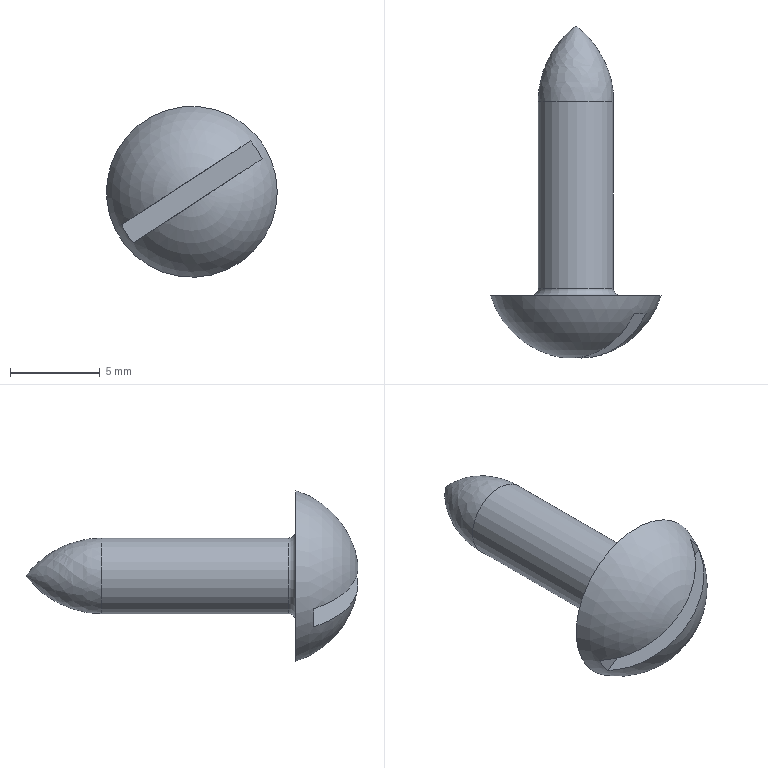Component | NX | 7_HALF_ROUND_SCREW_M5X15 | 1 solid | 8 faces | box 9.5 x 18.46 x 9.5 mm | volume 312 mm3 | plane 4 | sphere 1 | cylinder 1 | spline 1 | torus 1 | commonest cylinder face diameters 4.2 x1
STEP:
#1=CARTESIAN_POINT('',(0.,0.,0.));
#2=DIRECTION('',(0.,0.,1.));
#3=DIRECTION('',(1.,0.,0.));
#4=AXIS2_PLACEMENT_3D('',#1,#2,#3);
#5=CARTESIAN_POINT('',(-55.107,-157.206,-235.621));
#6=VERTEX_POINT('',#5);
#7=CARTESIAN_POINT('',(-55.507,-157.206,-235.093));
#8=VERTEX_POINT('',#7);
#9=CARTESIAN_POINT('',(-59.084,-157.206,-238.219));
#10=DIRECTION('',(0.,-1.,0.));
#11=DIRECTION('',(0.8372,0.,0.5469));
#12=AXIS2_PLACEMENT_3D('',#9,#10,#11);
#13=CIRCLE('',#12,4.75);
#14=CARTESIAN_POINT('',(-59.084,-155.733,-238.219));
#15=DIRECTION('',(0.,-1.,0.));
#16=DIRECTION('',(-0.5469,0.,0.8372));
#17=AXIS2_PLACEMENT_3D('',#14,#15,#16);
#18=SPHERICAL_SURFACE('',#17,4.973);
#19=CARTESIAN_POINT('',(10.996,0.3007));
#20=CARTESIAN_POINT('',(11.091,0.3007));
#21=CARTESIAN_POINT('',(11.281,0.3007));
#22=CARTESIAN_POINT('',(11.567,0.3007));
#23=CARTESIAN_POINT('',(11.852,0.3007));
#24=CARTESIAN_POINT('',(12.138,0.3007));
#25=CARTESIAN_POINT('',(12.424,0.3007));
#26=CARTESIAN_POINT('',(12.709,0.3007));
#27=CARTESIAN_POINT('',(12.995,0.3007));
#28=CARTESIAN_POINT('',(13.28,0.3007));
#29=CARTESIAN_POINT('',(13.566,0.3007));
#30=CARTESIAN_POINT('',(13.852,0.3007));
#31=CARTESIAN_POINT('',(14.137,0.3007));
#32=CARTESIAN_POINT('',(14.423,0.3007));
#33=CARTESIAN_POINT('',(14.708,0.3007));
#34=CARTESIAN_POINT('',(14.994,0.3007));
#35=CARTESIAN_POINT('',(15.28,0.3007));
#36=CARTESIAN_POINT('',(15.565,0.3007));
#37=CARTESIAN_POINT('',(15.851,0.3007));
#38=CARTESIAN_POINT('',(16.136,0.3007));
#39=CARTESIAN_POINT('',(16.422,0.3007));
#40=CARTESIAN_POINT('',(16.708,0.3007));
#41=CARTESIAN_POINT('',(16.993,0.3007));
#42=CARTESIAN_POINT('',(17.184,0.3007));
#43=CARTESIAN_POINT('',(17.279,0.3007));
#44=B_SPLINE_CURVE_WITH_KNOTS('',3,(#19,#20,#21,#22,#23,#24,#25,#26,#27,#28,#29,#30,#31,#32,#33,#34,#35,#36,#37,#38,#39,#40,#41,#42,#43),.UNSPECIFIED.,.F.,.F.,(4,1,1,1,1,1,1,1,1,1,1,1,1,1,1,1,1,1,1,1,1,1,4),(0.,0.2856,0.5712,0.8568,1.142,1.428,1.714,1.999,2.285,2.57,2.856,3.142,3.427,3.713,3.998,4.284,4.57,4.855,5.141,5.426,5.712,5.998,6.283),.QUASI_UNIFORM_KNOTS.);
#45=(GEOMETRIC_REPRESENTATION_CONTEXT(2)PARAMETRIC_REPRESENTATION_CONTEXT()REPRESENTATION_CONTEXT('',''));
#46=DEFINITIONAL_REPRESENTATION('',(#44),#45);
#47=PCURVE('',#18,#46);
#48=CARTESIAN_POINT('',(-60.232,-157.206,-236.461));
#49=DIRECTION('',(0.,-1.,0.));
#50=DIRECTION('',(0.8372,0.,0.5469));
#51=AXIS2_PLACEMENT_3D('',#48,#49,#50);
#52=PLANE('',#51);
#53=CARTESIAN_POINT('',(-0.,-2.1));
#54=DIRECTION('',(1.,-0.));
#55=AXIS2_PLACEMENT_2D('',#53,#54);
#56=CIRCLE('',#55,4.75);
#57=(GEOMETRIC_REPRESENTATION_CONTEXT(2)PARAMETRIC_REPRESENTATION_CONTEXT()REPRESENTATION_CONTEXT('',''));
#58=DEFINITIONAL_REPRESENTATION('',(#56),#57);
#59=PCURVE('',#52,#58);
#60=SURFACE_CURVE('',#13,(#47,#59),.PCURVE_S1.);
#61=EDGE_CURVE('',#6,#8,#60,.T.);
#62=ORIENTED_EDGE('',*,*,#61,.T.);
#63=CARTESIAN_POINT('',(-55.835,-158.206,-235.38));
#64=VERTEX_POINT('',#63);
#65=CARTESIAN_POINT('',(-55.507,-157.206,-235.093));
#66=CARTESIAN_POINT('',(-55.568,-157.467,-235.147));
#67=CARTESIAN_POINT('',(-55.643,-157.722,-235.212));
#68=CARTESIAN_POINT('',(-55.733,-157.969,-235.29));
#69=CARTESIAN_POINT('',(-55.835,-158.206,-235.38));
#70=B_SPLINE_CURVE_WITH_KNOTS('',4,(#65,#66,#67,#68,#69),.UNSPECIFIED.,.F.,.F.,(5,5),(0.3007,0.5205),.PIECEWISE_BEZIER_KNOTS.);
#71=CARTESIAN_POINT('',(11.135,0.));
#72=DIRECTION('',(0.,1.));
#73=VECTOR('',#72,1.);
#74=LINE('',#71,#73);
#75=(GEOMETRIC_REPRESENTATION_CONTEXT(2)PARAMETRIC_REPRESENTATION_CONTEXT()REPRESENTATION_CONTEXT('',''));
#76=DEFINITIONAL_REPRESENTATION('',(#74),#75);
#77=PCURVE('',#18,#76);
#78=CARTESIAN_POINT('',(4.852,0.));
#79=DIRECTION('',(0.,1.));
#80=VECTOR('',#79,1.);
#81=LINE('',#78,#80);
#82=(GEOMETRIC_REPRESENTATION_CONTEXT(2)PARAMETRIC_REPRESENTATION_CONTEXT()REPRESENTATION_CONTEXT('',''));
#83=DEFINITIONAL_REPRESENTATION('',(#81),#82);
#84=PCURVE('',#18,#83);
#85=SEAM_CURVE('',#70,(#77,#84),.PCURVE_S1.);
#86=EDGE_CURVE('',#8,#64,#85,.T.);
#87=ORIENTED_EDGE('',*,*,#86,.T.);
#88=CARTESIAN_POINT('',(-55.179,-158.206,-236.384));
#89=VERTEX_POINT('',#88);
#90=CARTESIAN_POINT('',(-59.084,-158.206,-238.219));
#91=DIRECTION('',(0.,-1.,0.));
#92=DIRECTION('',(0.8372,0.,0.5469));
#93=AXIS2_PLACEMENT_3D('',#90,#91,#92);
#94=CIRCLE('',#93,4.315);
#95=CARTESIAN_POINT('',(4.712,0.5205));
#96=DIRECTION('',(1.,0.));
#97=VECTOR('',#96,1.);
#98=LINE('',#95,#97);
#99=(GEOMETRIC_REPRESENTATION_CONTEXT(2)PARAMETRIC_REPRESENTATION_CONTEXT()REPRESENTATION_CONTEXT('',''));
#100=DEFINITIONAL_REPRESENTATION('',(#98),#99);
#101=PCURVE('',#18,#100);
#102=CARTESIAN_POINT('',(-51.131,-158.206,-233.023));
#103=DIRECTION('',(0.,-1.,0.));
#104=DIRECTION('',(0.8372,0.,0.5469));
#105=AXIS2_PLACEMENT_3D('',#102,#103,#104);
#106=PLANE('',#105);
#107=CARTESIAN_POINT('',(-9.5,-0.));
#108=DIRECTION('',(1.,-0.));
#109=AXIS2_PLACEMENT_2D('',#107,#108);
#110=CIRCLE('',#109,4.315);
#111=(GEOMETRIC_REPRESENTATION_CONTEXT(2)PARAMETRIC_REPRESENTATION_CONTEXT()REPRESENTATION_CONTEXT('',''));
#112=DEFINITIONAL_REPRESENTATION('',(#110),#111);
#113=PCURVE('',#106,#112);
#114=SURFACE_CURVE('',#94,(#101,#113),.PCURVE_S1.);
#115=EDGE_CURVE('',#89,#64,#114,.T.);
#116=ORIENTED_EDGE('',*,*,#115,.F.);
#117=CARTESIAN_POINT('',(-62.333,-158.206,-241.058));
#118=VERTEX_POINT('',#117);
#119=CARTESIAN_POINT('',(-58.756,-155.733,-238.721));
#120=DIRECTION('',(-0.5469,0.,0.8372));
#121=DIRECTION('',(-0.,-1.,0.));
#122=AXIS2_PLACEMENT_3D('',#119,#120,#121);
#123=CIRCLE('',#122,4.937);
#124=CARTESIAN_POINT('',(7.993,0.5205));
#125=CARTESIAN_POINT('',(7.996,0.5519));
#126=CARTESIAN_POINT('',(8.002,0.6146));
#127=CARTESIAN_POINT('',(8.013,0.7086));
#128=CARTESIAN_POINT('',(8.028,0.8024));
#129=CARTESIAN_POINT('',(8.047,0.8959));
#130=CARTESIAN_POINT('',(8.074,0.989));
#131=CARTESIAN_POINT('',(8.111,1.081));
#132=CARTESIAN_POINT('',(8.165,1.173));
#133=CARTESIAN_POINT('',(8.25,1.262));
#134=CARTESIAN_POINT('',(8.404,1.347));
#135=CARTESIAN_POINT('',(8.685,1.423));
#136=CARTESIAN_POINT('',(9.425,1.463));
#137=CARTESIAN_POINT('',(10.164,1.423));
#138=CARTESIAN_POINT('',(10.445,1.347));
#139=CARTESIAN_POINT('',(10.6,1.262));
#140=CARTESIAN_POINT('',(10.684,1.173));
#141=CARTESIAN_POINT('',(10.739,1.081));
#142=CARTESIAN_POINT('',(10.776,0.989));
#143=CARTESIAN_POINT('',(10.802,0.8959));
#144=CARTESIAN_POINT('',(10.822,0.8024));
#145=CARTESIAN_POINT('',(10.837,0.7086));
#146=CARTESIAN_POINT('',(10.848,0.6146));
#147=CARTESIAN_POINT('',(10.854,0.5519));
#148=CARTESIAN_POINT('',(10.856,0.5205));
#149=B_SPLINE_CURVE_WITH_KNOTS('',3,(#124,#125,#126,#127,#128,#129,#130,#131,#132,#133,#134,#135,#136,#137,#138,#139,#140,#141,#142,#143,#144,#145,#146,#147,#148),.UNSPECIFIED.,.F.,.F.,(4,1,1,1,1,1,1,1,1,1,1,1,1,1,1,1,1,1,1,1,1,1,4),(5.237,5.332,5.427,5.522,5.617,5.713,5.808,5.903,5.998,6.093,6.188,6.283,6.378,6.473,6.568,6.664,6.759,6.854,6.949,7.044,7.139,7.234,7.329),.QUASI_UNIFORM_KNOTS.);
#150=(GEOMETRIC_REPRESENTATION_CONTEXT(2)PARAMETRIC_REPRESENTATION_CONTEXT()REPRESENTATION_CONTEXT('',''));
#151=DEFINITIONAL_REPRESENTATION('',(#149),#150);
#152=PCURVE('',#18,#151);
#153=CARTESIAN_POINT('',(-50.803,-160.706,-233.525));
#154=DIRECTION('',(-0.5469,0.,0.8372));
#155=DIRECTION('',(-0.,-1.,0.));
#156=AXIS2_PLACEMENT_3D('',#153,#154,#155);
#157=PLANE('',#156);
#158=CARTESIAN_POINT('',(-4.973,-9.5));
#159=DIRECTION('',(1.,-0.));
#160=AXIS2_PLACEMENT_2D('',#158,#159);
#161=CIRCLE('',#160,4.937);
#162=(GEOMETRIC_REPRESENTATION_CONTEXT(2)PARAMETRIC_REPRESENTATION_CONTEXT()REPRESENTATION_CONTEXT('',''));
#163=DEFINITIONAL_REPRESENTATION('',(#161),#162);
#164=PCURVE('',#157,#163);
#165=SURFACE_CURVE('',#123,(#152,#164),.PCURVE_S1.);
#166=EDGE_CURVE('',#118,#89,#165,.T.);
#167=ORIENTED_EDGE('',*,*,#166,.F.);
#168=CARTESIAN_POINT('',(-62.989,-158.206,-240.054));
#169=VERTEX_POINT('',#168);
#170=CARTESIAN_POINT('',(-59.084,-158.206,-238.219));
#171=DIRECTION('',(0.,-1.,0.));
#172=DIRECTION('',(0.8372,0.,0.5469));
#173=AXIS2_PLACEMENT_3D('',#170,#171,#172);
#174=CIRCLE('',#173,4.315);
#175=CARTESIAN_POINT('',(4.712,0.5205));
#176=DIRECTION('',(1.,-0.));
#177=VECTOR('',#176,1.);
#178=LINE('',#175,#177);
#179=(GEOMETRIC_REPRESENTATION_CONTEXT(2)PARAMETRIC_REPRESENTATION_CONTEXT()REPRESENTATION_CONTEXT('',''));
#180=DEFINITIONAL_REPRESENTATION('',(#178),#179);
#181=PCURVE('',#18,#180);
#182=CARTESIAN_POINT('',(-9.5,-0.));
#183=DIRECTION('',(1.,-0.));
#184=AXIS2_PLACEMENT_2D('',#182,#183);
#185=CIRCLE('',#184,4.315);
#186=(GEOMETRIC_REPRESENTATION_CONTEXT(2)PARAMETRIC_REPRESENTATION_CONTEXT()REPRESENTATION_CONTEXT('',''));
#187=DEFINITIONAL_REPRESENTATION('',(#185),#186);
#188=PCURVE('',#106,#187);
#189=SURFACE_CURVE('',#174,(#181,#188),.PCURVE_S1.);
#190=EDGE_CURVE('',#169,#118,#189,.T.);
#191=ORIENTED_EDGE('',*,*,#190,.F.);
#192=CARTESIAN_POINT('',(-59.412,-155.733,-237.717));
#193=DIRECTION('',(0.5469,0.,-0.8372));
#194=DIRECTION('',(-0.,1.,0.));
#195=AXIS2_PLACEMENT_3D('',#192,#193,#194);
#196=CIRCLE('',#195,4.937);
#197=CARTESIAN_POINT('',(4.852,0.5205));
#198=CARTESIAN_POINT('',(4.854,0.5519));
#199=CARTESIAN_POINT('',(4.86,0.6146));
#200=CARTESIAN_POINT('',(4.871,0.7086));
#201=CARTESIAN_POINT('',(4.886,0.8024));
#202=CARTESIAN_POINT('',(4.906,0.8959));
#203=CARTESIAN_POINT('',(4.932,0.989));
#204=CARTESIAN_POINT('',(4.969,1.081));
#205=CARTESIAN_POINT('',(5.024,1.173));
#206=CARTESIAN_POINT('',(5.108,1.262));
#207=CARTESIAN_POINT('',(5.263,1.347));
#208=CARTESIAN_POINT('',(5.543,1.423));
#209=CARTESIAN_POINT('',(6.283,1.463));
#210=CARTESIAN_POINT('',(7.023,1.423));
#211=CARTESIAN_POINT('',(7.304,1.347));
#212=CARTESIAN_POINT('',(7.458,1.262));
#213=CARTESIAN_POINT('',(7.543,1.173));
#214=CARTESIAN_POINT('',(7.597,1.081));
#215=CARTESIAN_POINT('',(7.634,0.989));
#216=CARTESIAN_POINT('',(7.661,0.8959));
#217=CARTESIAN_POINT('',(7.68,0.8024));
#218=CARTESIAN_POINT('',(7.695,0.7086));
#219=CARTESIAN_POINT('',(7.706,0.6146));
#220=CARTESIAN_POINT('',(7.712,0.5519));
#221=CARTESIAN_POINT('',(7.714,0.5205));
#222=B_SPLINE_CURVE_WITH_KNOTS('',3,(#197,#198,#199,#200,#201,#202,#203,#204,#205,#206,#207,#208,#209,#210,#211,#212,#213,#214,#215,#216,#217,#218,#219,#220,#221),.UNSPECIFIED.,.F.,.F.,(4,1,1,1,1,1,1,1,1,1,1,1,1,1,1,1,1,1,1,1,1,1,4),(2.096,2.191,2.286,2.381,2.476,2.571,2.666,2.761,2.856,2.951,3.046,3.142,3.237,3.332,3.427,3.522,3.617,3.712,3.807,3.902,3.997,4.093,4.188),.QUASI_UNIFORM_KNOTS.);
#223=(GEOMETRIC_REPRESENTATION_CONTEXT(2)PARAMETRIC_REPRESENTATION_CONTEXT()REPRESENTATION_CONTEXT('',''));
#224=DEFINITIONAL_REPRESENTATION('',(#222),#223);
#225=PCURVE('',#18,#224);
#226=CARTESIAN_POINT('',(-51.459,-158.206,-232.521));
#227=DIRECTION('',(0.5469,0.,-0.8372));
#228=DIRECTION('',(-0.,1.,0.));
#229=AXIS2_PLACEMENT_3D('',#226,#227,#228);
#230=PLANE('',#229);
#231=CARTESIAN_POINT('',(2.473,-9.5));
#232=DIRECTION('',(1.,-0.));
#233=AXIS2_PLACEMENT_2D('',#231,#232);
#234=CIRCLE('',#233,4.937);
#235=(GEOMETRIC_REPRESENTATION_CONTEXT(2)PARAMETRIC_REPRESENTATION_CONTEXT()REPRESENTATION_CONTEXT('',''));
#236=DEFINITIONAL_REPRESENTATION('',(#234),#235);
#237=PCURVE('',#230,#236);
#238=SURFACE_CURVE('',#196,(#225,#237),.PCURVE_S1.);
#239=EDGE_CURVE('',#64,#169,#238,.T.);
#240=ORIENTED_EDGE('',*,*,#239,.F.);
#241=ORIENTED_EDGE('',*,*,#86,.F.);
#242=CARTESIAN_POINT('',(-59.084,-157.206,-238.219));
#243=DIRECTION('',(0.,-1.,0.));
#244=DIRECTION('',(0.8372,0.,0.5469));
#245=AXIS2_PLACEMENT_3D('',#242,#243,#244);
#246=CIRCLE('',#245,4.75);
#247=CARTESIAN_POINT('',(4.712,0.3007));
#248=CARTESIAN_POINT('',(4.808,0.3007));
#249=CARTESIAN_POINT('',(4.998,0.3007));
#250=CARTESIAN_POINT('',(5.284,0.3007));
#251=CARTESIAN_POINT('',(5.569,0.3007));
#252=CARTESIAN_POINT('',(5.855,0.3007));
#253=CARTESIAN_POINT('',(6.14,0.3007));
#254=CARTESIAN_POINT('',(6.426,0.3007));
#255=CARTESIAN_POINT('',(6.712,0.3007));
#256=CARTESIAN_POINT('',(6.997,0.3007));
#257=CARTESIAN_POINT('',(7.283,0.3007));
#258=CARTESIAN_POINT('',(7.568,0.3007));
#259=CARTESIAN_POINT('',(7.854,0.3007));
#260=CARTESIAN_POINT('',(8.14,0.3007));
#261=CARTESIAN_POINT('',(8.425,0.3007));
#262=CARTESIAN_POINT('',(8.711,0.3007));
#263=CARTESIAN_POINT('',(8.996,0.3007));
#264=CARTESIAN_POINT('',(9.282,0.3007));
#265=CARTESIAN_POINT('',(9.568,0.3007));
#266=CARTESIAN_POINT('',(9.853,0.3007));
#267=CARTESIAN_POINT('',(10.139,0.3007));
#268=CARTESIAN_POINT('',(10.424,0.3007));
#269=CARTESIAN_POINT('',(10.71,0.3007));
#270=CARTESIAN_POINT('',(10.9,0.3007));
#271=CARTESIAN_POINT('',(10.996,0.3007));
#272=B_SPLINE_CURVE_WITH_KNOTS('',3,(#247,#248,#249,#250,#251,#252,#253,#254,#255,#256,#257,#258,#259,#260,#261,#262,#263,#264,#265,#266,#267,#268,#269,#270,#271),.UNSPECIFIED.,.F.,.F.,(4,1,1,1,1,1,1,1,1,1,1,1,1,1,1,1,1,1,1,1,1,1,4),(0.,0.2856,0.5712,0.8568,1.142,1.428,1.714,1.999,2.285,2.57,2.856,3.142,3.427,3.713,3.998,4.284,4.57,4.855,5.141,5.426,5.712,5.998,6.283),.QUASI_UNIFORM_KNOTS.);
#273=(GEOMETRIC_REPRESENTATION_CONTEXT(2)PARAMETRIC_REPRESENTATION_CONTEXT()REPRESENTATION_CONTEXT('',''));
#274=DEFINITIONAL_REPRESENTATION('',(#272),#273);
#275=PCURVE('',#18,#274);
#276=CARTESIAN_POINT('',(-0.,-2.1));
#277=DIRECTION('',(1.,-0.));
#278=AXIS2_PLACEMENT_2D('',#276,#277);
#279=CIRCLE('',#278,4.75);
#280=(GEOMETRIC_REPRESENTATION_CONTEXT(2)PARAMETRIC_REPRESENTATION_CONTEXT()REPRESENTATION_CONTEXT('',''));
#281=DEFINITIONAL_REPRESENTATION('',(#279),#280);
#282=PCURVE('',#52,#281);
#283=SURFACE_CURVE('',#246,(#275,#282),.PCURVE_S1.);
#284=EDGE_CURVE('',#8,#6,#283,.T.);
#285=ORIENTED_EDGE('',*,*,#284,.T.);
#286=EDGE_LOOP('',(#62,#87,#116,#167,#191,#240,#241,#285));
#287=FACE_BOUND('',#286,.T.);
#288=ADVANCED_FACE('',(#287),#18,.T.);
#289=CARTESIAN_POINT('',(-56.991,-157.206,-236.852));
#290=VERTEX_POINT('',#289);
#291=CARTESIAN_POINT('',(-59.084,-157.206,-238.219));
#292=DIRECTION('',(0.,-1.,0.));
#293=DIRECTION('',(0.8372,0.,0.5469));
#294=AXIS2_PLACEMENT_3D('',#291,#292,#293);
#295=CIRCLE('',#294,2.5);
#296=CARTESIAN_POINT('',(-0.,-2.1));
#297=DIRECTION('',(1.,-0.));
#298=AXIS2_PLACEMENT_2D('',#296,#297);
#299=CIRCLE('',#298,2.5);
#300=(GEOMETRIC_REPRESENTATION_CONTEXT(2)PARAMETRIC_REPRESENTATION_CONTEXT()REPRESENTATION_CONTEXT('',''));
#301=DEFINITIONAL_REPRESENTATION('',(#299),#300);
#302=PCURVE('',#52,#301);
#303=CARTESIAN_POINT('',(-59.084,-156.806,-238.219));
#304=DIRECTION('',(0.,-1.,0.));
#305=DIRECTION('',(0.8372,0.,0.5469));
#306=AXIS2_PLACEMENT_3D('',#303,#304,#305);
#307=TOROIDAL_SURFACE('',#306,2.5,0.4);
#308=CARTESIAN_POINT('',(0.,7.854));
#309=DIRECTION('',(1.,-0.));
#310=VECTOR('',#309,1.);
#311=LINE('',#308,#310);
#312=(GEOMETRIC_REPRESENTATION_CONTEXT(2)PARAMETRIC_REPRESENTATION_CONTEXT()REPRESENTATION_CONTEXT('',''));
#313=DEFINITIONAL_REPRESENTATION('',(#311),#312);
#314=PCURVE('',#307,#313);
#315=SURFACE_CURVE('',#295,(#302,#314),.PCURVE_S1.);
#316=EDGE_CURVE('',#290,#290,#315,.T.);
#317=ORIENTED_EDGE('',*,*,#316,.T.);
#318=EDGE_LOOP('',(#317));
#319=FACE_BOUND('',#318,.T.);
#320=ORIENTED_EDGE('',*,*,#61,.F.);
#321=ORIENTED_EDGE('',*,*,#284,.F.);
#322=EDGE_LOOP('',(#320,#321));
#323=FACE_BOUND('',#322,.T.);
#324=ADVANCED_FACE('',(#319,#323),#52,.F.);
#325=CARTESIAN_POINT('',(-57.326,-156.806,-237.07));
#326=VERTEX_POINT('',#325);
#327=CARTESIAN_POINT('',(-59.084,-156.806,-238.219));
#328=DIRECTION('',(0.,1.,0.));
#329=DIRECTION('',(0.8372,0.,0.5469));
#330=AXIS2_PLACEMENT_3D('',#327,#328,#329);
#331=CIRCLE('',#330,2.1);
#332=CARTESIAN_POINT('',(-59.084,-157.206,-238.219));
#333=DIRECTION('',(0.,-1.,0.));
#334=DIRECTION('',(0.8372,0.,0.5469));
#335=AXIS2_PLACEMENT_3D('',#332,#333,#334);
#336=CYLINDRICAL_SURFACE('',#335,2.1);
#337=CARTESIAN_POINT('',(6.283,-0.4));
#338=DIRECTION('',(-1.,0.));
#339=VECTOR('',#338,1.);
#340=LINE('',#337,#339);
#341=(GEOMETRIC_REPRESENTATION_CONTEXT(2)PARAMETRIC_REPRESENTATION_CONTEXT()REPRESENTATION_CONTEXT('',''));
#342=DEFINITIONAL_REPRESENTATION('',(#340),#341);
#343=PCURVE('',#336,#342);
#344=CARTESIAN_POINT('',(6.283,9.425));
#345=DIRECTION('',(-1.,0.));
#346=VECTOR('',#345,1.);
#347=LINE('',#344,#346);
#348=(GEOMETRIC_REPRESENTATION_CONTEXT(2)PARAMETRIC_REPRESENTATION_CONTEXT()REPRESENTATION_CONTEXT('',''));
#349=DEFINITIONAL_REPRESENTATION('',(#347),#348);
#350=PCURVE('',#307,#349);
#351=SURFACE_CURVE('',#331,(#343,#350),.PCURVE_S1.);
#352=EDGE_CURVE('',#326,#326,#351,.T.);
#353=ORIENTED_EDGE('',*,*,#352,.T.);
#354=CARTESIAN_POINT('',(-57.326,-146.406,-237.07));
#355=VERTEX_POINT('',#354);
#356=CARTESIAN_POINT('',(-57.326,-146.406,-237.07));
#357=CARTESIAN_POINT('',(-57.326,-156.806,-237.07));
#358=B_SPLINE_CURVE_WITH_KNOTS('',1,(#356,#357),.UNSPECIFIED.,.F.,.F.,(2,2),(-10.8,-0.4),.PIECEWISE_BEZIER_KNOTS.);
#359=CARTESIAN_POINT('',(0.,0.));
#360=DIRECTION('',(0.,1.));
#361=VECTOR('',#360,1.);
#362=LINE('',#359,#361);
#363=(GEOMETRIC_REPRESENTATION_CONTEXT(2)PARAMETRIC_REPRESENTATION_CONTEXT()REPRESENTATION_CONTEXT('',''));
#364=DEFINITIONAL_REPRESENTATION('',(#362),#363);
#365=PCURVE('',#336,#364);
#366=CARTESIAN_POINT('',(6.283,0.));
#367=DIRECTION('',(0.,1.));
#368=VECTOR('',#367,1.);
#369=LINE('',#366,#368);
#370=(GEOMETRIC_REPRESENTATION_CONTEXT(2)PARAMETRIC_REPRESENTATION_CONTEXT()REPRESENTATION_CONTEXT('',''));
#371=DEFINITIONAL_REPRESENTATION('',(#369),#370);
#372=PCURVE('',#336,#371);
#373=SEAM_CURVE('',#358,(#365,#372),.PCURVE_S1.);
#374=EDGE_CURVE('',#355,#326,#373,.T.);
#375=ORIENTED_EDGE('',*,*,#374,.F.);
#376=CARTESIAN_POINT('',(-59.084,-146.406,-238.219));
#377=DIRECTION('',(0.,-1.,0.));
#378=DIRECTION('',(0.8372,0.,0.5469));
#379=AXIS2_PLACEMENT_3D('',#376,#377,#378);
#380=CIRCLE('',#379,2.1);
#381=CARTESIAN_POINT('',(0.,-10.8));
#382=DIRECTION('',(1.,0.));
#383=VECTOR('',#382,1.);
#384=LINE('',#381,#383);
#385=(GEOMETRIC_REPRESENTATION_CONTEXT(2)PARAMETRIC_REPRESENTATION_CONTEXT()REPRESENTATION_CONTEXT('',''));
#386=DEFINITIONAL_REPRESENTATION('',(#384),#385);
#387=PCURVE('',#336,#386);
#388=CARTESIAN_POINT('',(-57.326,-146.406,-237.07));
#389=CARTESIAN_POINT('',(-59.623,-146.406,-233.554));
#390=CARTESIAN_POINT('',(-63.139,-146.406,-235.852));
#391=CARTESIAN_POINT('',(-60.842,-146.406,-239.368));
#392=CARTESIAN_POINT('',(-58.545,-146.406,-242.884));
#393=CARTESIAN_POINT('',(-55.029,-146.406,-240.587));
#394=CARTESIAN_POINT('',(-57.326,-146.406,-237.07));
#395=CARTESIAN_POINT('',(-57.326,-144.723,-237.07));
#396=CARTESIAN_POINT('',(-59.623,-144.723,-233.554));
#397=CARTESIAN_POINT('',(-63.139,-144.723,-235.852));
#398=CARTESIAN_POINT('',(-60.842,-144.723,-239.368));
#399=CARTESIAN_POINT('',(-58.545,-144.723,-242.884));
#400=CARTESIAN_POINT('',(-55.029,-144.723,-240.587));
#401=CARTESIAN_POINT('',(-57.326,-144.723,-237.07));
#402=CARTESIAN_POINT('',(-57.956,-143.217,-237.482));
#403=CARTESIAN_POINT('',(-59.43,-143.217,-235.227));
#404=CARTESIAN_POINT('',(-61.685,-143.217,-236.7));
#405=CARTESIAN_POINT('',(-60.211,-143.217,-238.956));
#406=CARTESIAN_POINT('',(-58.738,-143.217,-241.211));
#407=CARTESIAN_POINT('',(-56.483,-143.217,-239.738));
#408=CARTESIAN_POINT('',(-57.956,-143.217,-237.482));
#409=CARTESIAN_POINT('',(-59.084,-142.206,-238.219));
#410=CARTESIAN_POINT('',(-59.084,-142.206,-238.219));
#411=CARTESIAN_POINT('',(-59.084,-142.206,-238.219));
#412=CARTESIAN_POINT('',(-59.084,-142.206,-238.219));
#413=CARTESIAN_POINT('',(-59.084,-142.206,-238.219));
#414=CARTESIAN_POINT('',(-59.084,-142.206,-238.219));
#415=CARTESIAN_POINT('',(-59.084,-142.206,-238.219));
#416=(BOUNDED_SURFACE()B_SPLINE_SURFACE(3,3,((#388,#389,#390,#391,#392,#393,#394),(#395,#396,#397,#398,#399,#400,#401),(#402,#403,#404,#405,#406,#407,#408),(#409,#410,#411,#412,#413,#414,#415)),.UNSPECIFIED.,.F.,.T.,.F.)B_SPLINE_SURFACE_WITH_KNOTS((4,4),(1,3,3,3,1),(0.,1.),(-0.5,0.,0.5,1.,1.5),.UNSPECIFIED.)GEOMETRIC_REPRESENTATION_ITEM()RATIONAL_B_SPLINE_SURFACE(((1.,0.3333,0.3333,1.,0.3333,0.3333,1.),(0.9296,0.3099,0.3099,0.9296,0.3099,0.3099,0.9296),(0.9296,0.3099,0.3099,0.9296,0.3099,0.3099,0.9296),(1.,0.3333,0.3333,1.,0.3333,0.3333,1.)))REPRESENTATION_ITEM('')SURFACE());
#417=CARTESIAN_POINT('',(0.,0.));
#418=CARTESIAN_POINT('',(0.,0.02352));
#419=CARTESIAN_POINT('',(0.,0.06491));
#420=CARTESIAN_POINT('',(0.,0.1146));
#421=CARTESIAN_POINT('',(0.,0.1575));
#422=CARTESIAN_POINT('',(0.,0.196));
#423=CARTESIAN_POINT('',(0.,0.2322));
#424=CARTESIAN_POINT('',(0.,0.2678));
#425=CARTESIAN_POINT('',(0.,0.304));
#426=CARTESIAN_POINT('',(0.,0.3425));
#427=CARTESIAN_POINT('',(0.,0.3856));
#428=CARTESIAN_POINT('',(0.,0.4343));
#429=CARTESIAN_POINT('',(0.,0.5));
#430=CARTESIAN_POINT('',(0.,0.5657));
#431=CARTESIAN_POINT('',(0.,0.6144));
#432=CARTESIAN_POINT('',(0.,0.6575));
#433=CARTESIAN_POINT('',(0.,0.696));
#434=CARTESIAN_POINT('',(0.,0.7322));
#435=CARTESIAN_POINT('',(0.,0.7678));
#436=CARTESIAN_POINT('',(0.,0.804));
#437=CARTESIAN_POINT('',(0.,0.8425));
#438=CARTESIAN_POINT('',(0.,0.8854));
#439=CARTESIAN_POINT('',(0.,0.9351));
#440=CARTESIAN_POINT('',(0.,0.9765));
#441=CARTESIAN_POINT('',(0.,1.));
#442=B_SPLINE_CURVE_WITH_KNOTS('',3,(#417,#418,#419,#420,#421,#422,#423,#424,#425,#426,#427,#428,#429,#430,#431,#432,#433,#434,#435,#436,#437,#438,#439,#440,#441),.UNSPECIFIED.,.F.,.F.,(4,1,1,1,1,1,1,1,1,1,1,1,1,1,1,1,1,1,1,1,1,1,4),(0.,0.2856,0.5712,0.8568,1.142,1.428,1.714,1.999,2.285,2.57,2.856,3.142,3.427,3.713,3.998,4.284,4.57,4.855,5.141,5.426,5.712,5.998,6.283),.QUASI_UNIFORM_KNOTS.);
#443=(GEOMETRIC_REPRESENTATION_CONTEXT(2)PARAMETRIC_REPRESENTATION_CONTEXT()REPRESENTATION_CONTEXT('',''));
#444=DEFINITIONAL_REPRESENTATION('',(#442),#443);
#445=PCURVE('',#416,#444);
#446=SURFACE_CURVE('',#380,(#387,#445),.PCURVE_S1.);
#447=EDGE_CURVE('',#355,#355,#446,.T.);
#448=ORIENTED_EDGE('',*,*,#447,.T.);
#449=ORIENTED_EDGE('',*,*,#374,.T.);
#450=EDGE_LOOP('',(#353,#375,#448,#449));
#451=FACE_BOUND('',#450,.T.);
#452=ADVANCED_FACE('',(#451),#336,.T.);
#453=ORIENTED_EDGE('',*,*,#447,.F.);
#454=CARTESIAN_POINT('',(-59.084,-142.206,-238.219));
#455=VERTEX_POINT('',#454);
#456=CARTESIAN_POINT('',(-57.326,-146.406,-237.07));
#457=CARTESIAN_POINT('',(-57.326,-144.723,-237.07));
#458=CARTESIAN_POINT('',(-57.956,-143.217,-237.482));
#459=CARTESIAN_POINT('',(-59.084,-142.206,-238.219));
#460=(BOUNDED_CURVE()B_SPLINE_CURVE(3,(#456,#457,#458,#459),.UNSPECIFIED.,.F.,.F.)B_SPLINE_CURVE_WITH_KNOTS((4,4),(0.,1.),.PIECEWISE_BEZIER_KNOTS.)CURVE()GEOMETRIC_REPRESENTATION_ITEM()RATIONAL_B_SPLINE_CURVE((1.,0.9296,0.9296,1.))REPRESENTATION_ITEM(''));
#461=CARTESIAN_POINT('',(0.,0.));
#462=DIRECTION('',(1.,0.));
#463=VECTOR('',#462,1.);
#464=LINE('',#461,#463);
#465=(GEOMETRIC_REPRESENTATION_CONTEXT(2)PARAMETRIC_REPRESENTATION_CONTEXT()REPRESENTATION_CONTEXT('',''));
#466=DEFINITIONAL_REPRESENTATION('',(#464),#465);
#467=PCURVE('',#416,#466);
#468=CARTESIAN_POINT('',(0.,1.));
#469=DIRECTION('',(1.,0.));
#470=VECTOR('',#469,1.);
#471=LINE('',#468,#470);
#472=(GEOMETRIC_REPRESENTATION_CONTEXT(2)PARAMETRIC_REPRESENTATION_CONTEXT()REPRESENTATION_CONTEXT('',''));
#473=DEFINITIONAL_REPRESENTATION('',(#471),#472);
#474=PCURVE('',#416,#473);
#475=SEAM_CURVE('',#460,(#467,#474),.PCURVE_S1.);
#476=EDGE_CURVE('',#355,#455,#475,.T.);
#477=ORIENTED_EDGE('',*,*,#476,.T.);
#478=ORIENTED_EDGE('',*,*,#476,.F.);
#479=EDGE_LOOP('',(#453,#477,#478));
#480=FACE_BOUND('',#479,.T.);
#481=ADVANCED_FACE('',(#480),#416,.T.);
#482=ORIENTED_EDGE('',*,*,#166,.T.);
#483=CARTESIAN_POINT('',(-50.803,-158.206,-233.525));
#484=DIRECTION('',(-0.8372,0.,-0.5469));
#485=VECTOR('',#484,1.);
#486=LINE('',#483,#485);
#487=CARTESIAN_POINT('',(-2.5,0.));
#488=DIRECTION('',(-0.,-1.));
#489=VECTOR('',#488,1.);
#490=LINE('',#487,#489);
#491=(GEOMETRIC_REPRESENTATION_CONTEXT(2)PARAMETRIC_REPRESENTATION_CONTEXT()REPRESENTATION_CONTEXT('',''));
#492=DEFINITIONAL_REPRESENTATION('',(#490),#491);
#493=PCURVE('',#157,#492);
#494=CARTESIAN_POINT('',(-0.,-0.6));
#495=DIRECTION('',(-1.,0.));
#496=VECTOR('',#495,1.);
#497=LINE('',#494,#496);
#498=(GEOMETRIC_REPRESENTATION_CONTEXT(2)PARAMETRIC_REPRESENTATION_CONTEXT()REPRESENTATION_CONTEXT('',''));
#499=DEFINITIONAL_REPRESENTATION('',(#497),#498);
#500=PCURVE('',#106,#499);
#501=SURFACE_CURVE('',#486,(#493,#500),.PCURVE_S1.);
#502=EDGE_CURVE('',#89,#118,#501,.T.);
#503=ORIENTED_EDGE('',*,*,#502,.T.);
#504=EDGE_LOOP('',(#482,#503));
#505=FACE_BOUND('',#504,.T.);
#506=ADVANCED_FACE('',(#505),#157,.T.);
#507=ORIENTED_EDGE('',*,*,#190,.T.);
#508=ORIENTED_EDGE('',*,*,#502,.F.);
#509=ORIENTED_EDGE('',*,*,#115,.T.);
#510=CARTESIAN_POINT('',(-51.459,-158.206,-232.521));
#511=DIRECTION('',(-0.8372,0.,-0.5469));
#512=VECTOR('',#511,1.);
#513=LINE('',#510,#512);
#514=CARTESIAN_POINT('',(0.,0.6));
#515=DIRECTION('',(-1.,0.));
#516=VECTOR('',#515,1.);
#517=LINE('',#514,#516);
#518=(GEOMETRIC_REPRESENTATION_CONTEXT(2)PARAMETRIC_REPRESENTATION_CONTEXT()REPRESENTATION_CONTEXT('',''));
#519=DEFINITIONAL_REPRESENTATION('',(#517),#518);
#520=PCURVE('',#106,#519);
#521=CARTESIAN_POINT('',(0.,0.));
#522=DIRECTION('',(-0.,-1.));
#523=VECTOR('',#522,1.);
#524=LINE('',#521,#523);
#525=(GEOMETRIC_REPRESENTATION_CONTEXT(2)PARAMETRIC_REPRESENTATION_CONTEXT()REPRESENTATION_CONTEXT('',''));
#526=DEFINITIONAL_REPRESENTATION('',(#524),#525);
#527=PCURVE('',#230,#526);
#528=SURFACE_CURVE('',#513,(#520,#527),.PCURVE_S1.);
#529=EDGE_CURVE('',#64,#169,#528,.T.);
#530=ORIENTED_EDGE('',*,*,#529,.T.);
#531=EDGE_LOOP('',(#507,#508,#509,#530));
#532=FACE_BOUND('',#531,.T.);
#533=ADVANCED_FACE('',(#532),#106,.T.);
#534=ORIENTED_EDGE('',*,*,#239,.T.);
#535=ORIENTED_EDGE('',*,*,#529,.F.);
#536=EDGE_LOOP('',(#534,#535));
#537=FACE_BOUND('',#536,.T.);
#538=ADVANCED_FACE('',(#537),#230,.T.);
#539=ORIENTED_EDGE('',*,*,#352,.T.);
#540=CARTESIAN_POINT('',(-56.991,-157.206,-236.852));
#541=CARTESIAN_POINT('',(-57.08,-157.206,-236.91));
#542=CARTESIAN_POINT('',(-57.168,-157.172,-236.967));
#543=CARTESIAN_POINT('',(-57.243,-157.107,-237.016));
#544=CARTESIAN_POINT('',(-57.297,-157.017,-237.052));
#545=CARTESIAN_POINT('',(-57.326,-156.913,-237.07));
#546=CARTESIAN_POINT('',(-57.326,-156.806,-237.07));
#547=(BOUNDED_CURVE()B_SPLINE_CURVE(6,(#540,#541,#542,#543,#544,#545,#546),.UNSPECIFIED.,.F.,.F.)B_SPLINE_CURVE_WITH_KNOTS((7,7),(1.571,3.142),.PIECEWISE_BEZIER_KNOTS.)CURVE()GEOMETRIC_REPRESENTATION_ITEM()RATIONAL_B_SPLINE_CURVE((1.031,1.01,0.9979,0.994,0.9979,1.01,1.031))REPRESENTATION_ITEM(''));
#548=CARTESIAN_POINT('',(0.,6.283));
#549=DIRECTION('',(0.,1.));
#550=VECTOR('',#549,1.);
#551=LINE('',#548,#550);
#552=(GEOMETRIC_REPRESENTATION_CONTEXT(2)PARAMETRIC_REPRESENTATION_CONTEXT()REPRESENTATION_CONTEXT('',''));
#553=DEFINITIONAL_REPRESENTATION('',(#551),#552);
#554=PCURVE('',#307,#553);
#555=CARTESIAN_POINT('',(6.283,6.283));
#556=DIRECTION('',(0.,1.));
#557=VECTOR('',#556,1.);
#558=LINE('',#555,#557);
#559=(GEOMETRIC_REPRESENTATION_CONTEXT(2)PARAMETRIC_REPRESENTATION_CONTEXT()REPRESENTATION_CONTEXT('',''));
#560=DEFINITIONAL_REPRESENTATION('',(#558),#559);
#561=PCURVE('',#307,#560);
#562=SEAM_CURVE('',#547,(#554,#561),.PCURVE_S1.);
#563=EDGE_CURVE('',#290,#326,#562,.T.);
#564=ORIENTED_EDGE('',*,*,#563,.F.);
#565=ORIENTED_EDGE('',*,*,#316,.T.);
#566=ORIENTED_EDGE('',*,*,#563,.T.);
#567=EDGE_LOOP('',(#539,#564,#565,#566));
#568=FACE_BOUND('',#567,.F.);
#569=ADVANCED_FACE('',(#568),#307,.F.);
#570=CLOSED_SHELL('',(#288,#324,#452,#481,#506,#533,#538,#569));
#571=MANIFOLD_SOLID_BREP('',#570);
#572=(LENGTH_UNIT()NAMED_UNIT(*)SI_UNIT(.MILLI.,.METRE.));
#573=UNCERTAINTY_MEASURE_WITH_UNIT(LENGTH_MEASURE(0.000005),#572,'','');
#574=(NAMED_UNIT(*)PLANE_ANGLE_UNIT()SI_UNIT($,.RADIAN.));
#575=(NAMED_UNIT(*)SI_UNIT($,.STERADIAN.)SOLID_ANGLE_UNIT());
#576=(GEOMETRIC_REPRESENTATION_CONTEXT(3)GLOBAL_UNCERTAINTY_ASSIGNED_CONTEXT((#573))GLOBAL_UNIT_ASSIGNED_CONTEXT((#572,#574,#575))REPRESENTATION_CONTEXT('',''));
#577=ADVANCED_BREP_SHAPE_REPRESENTATION('',(#4,#571),#576);